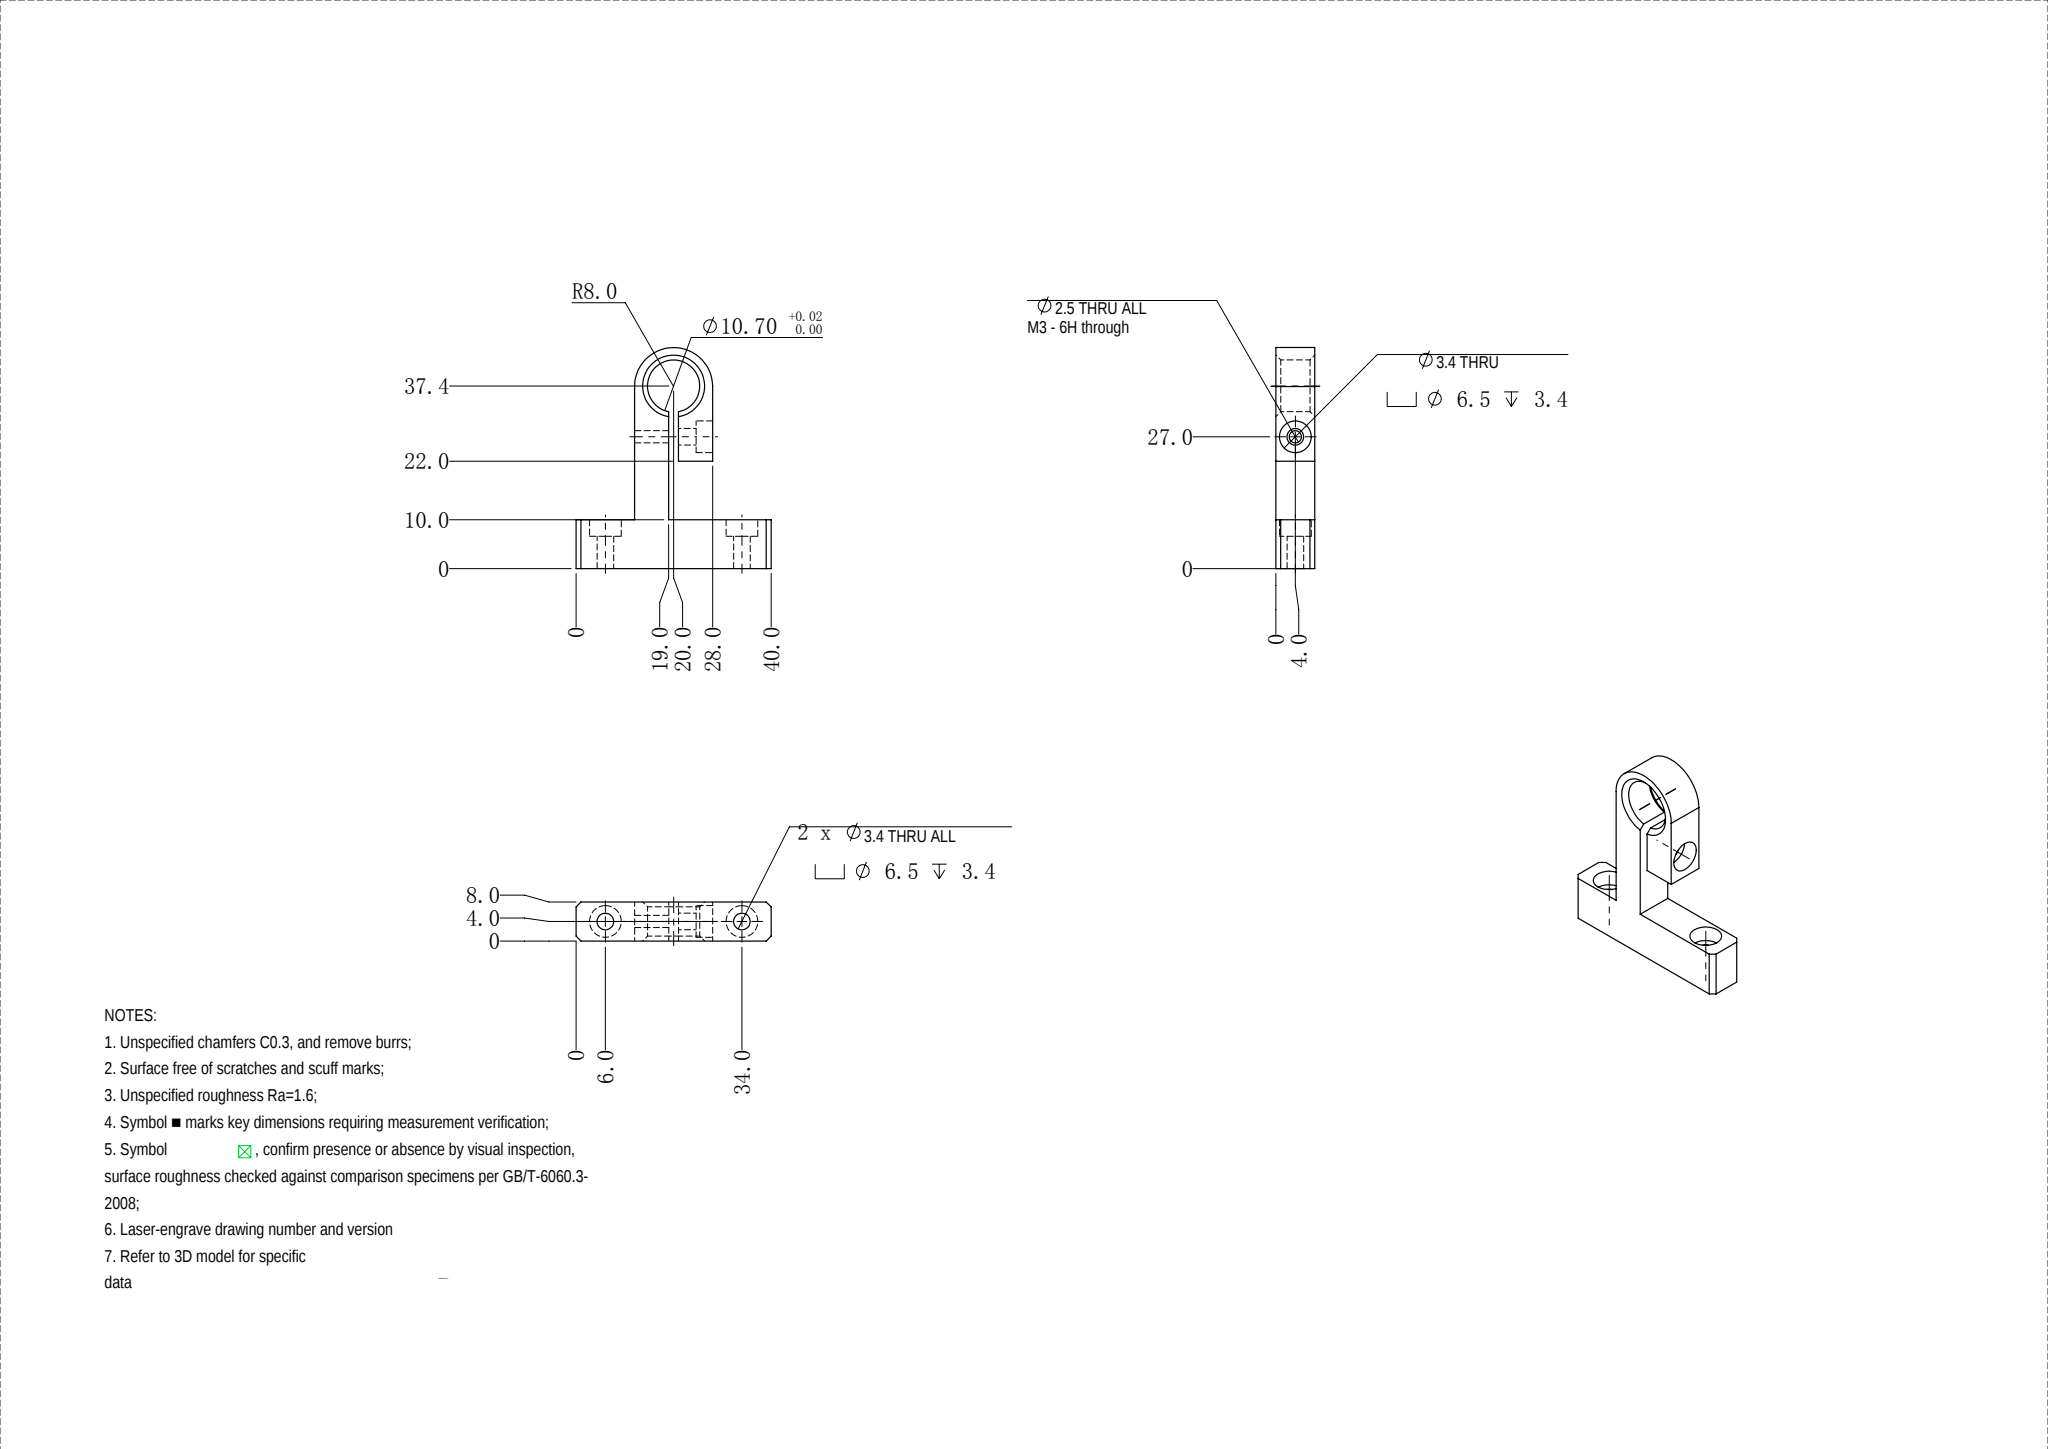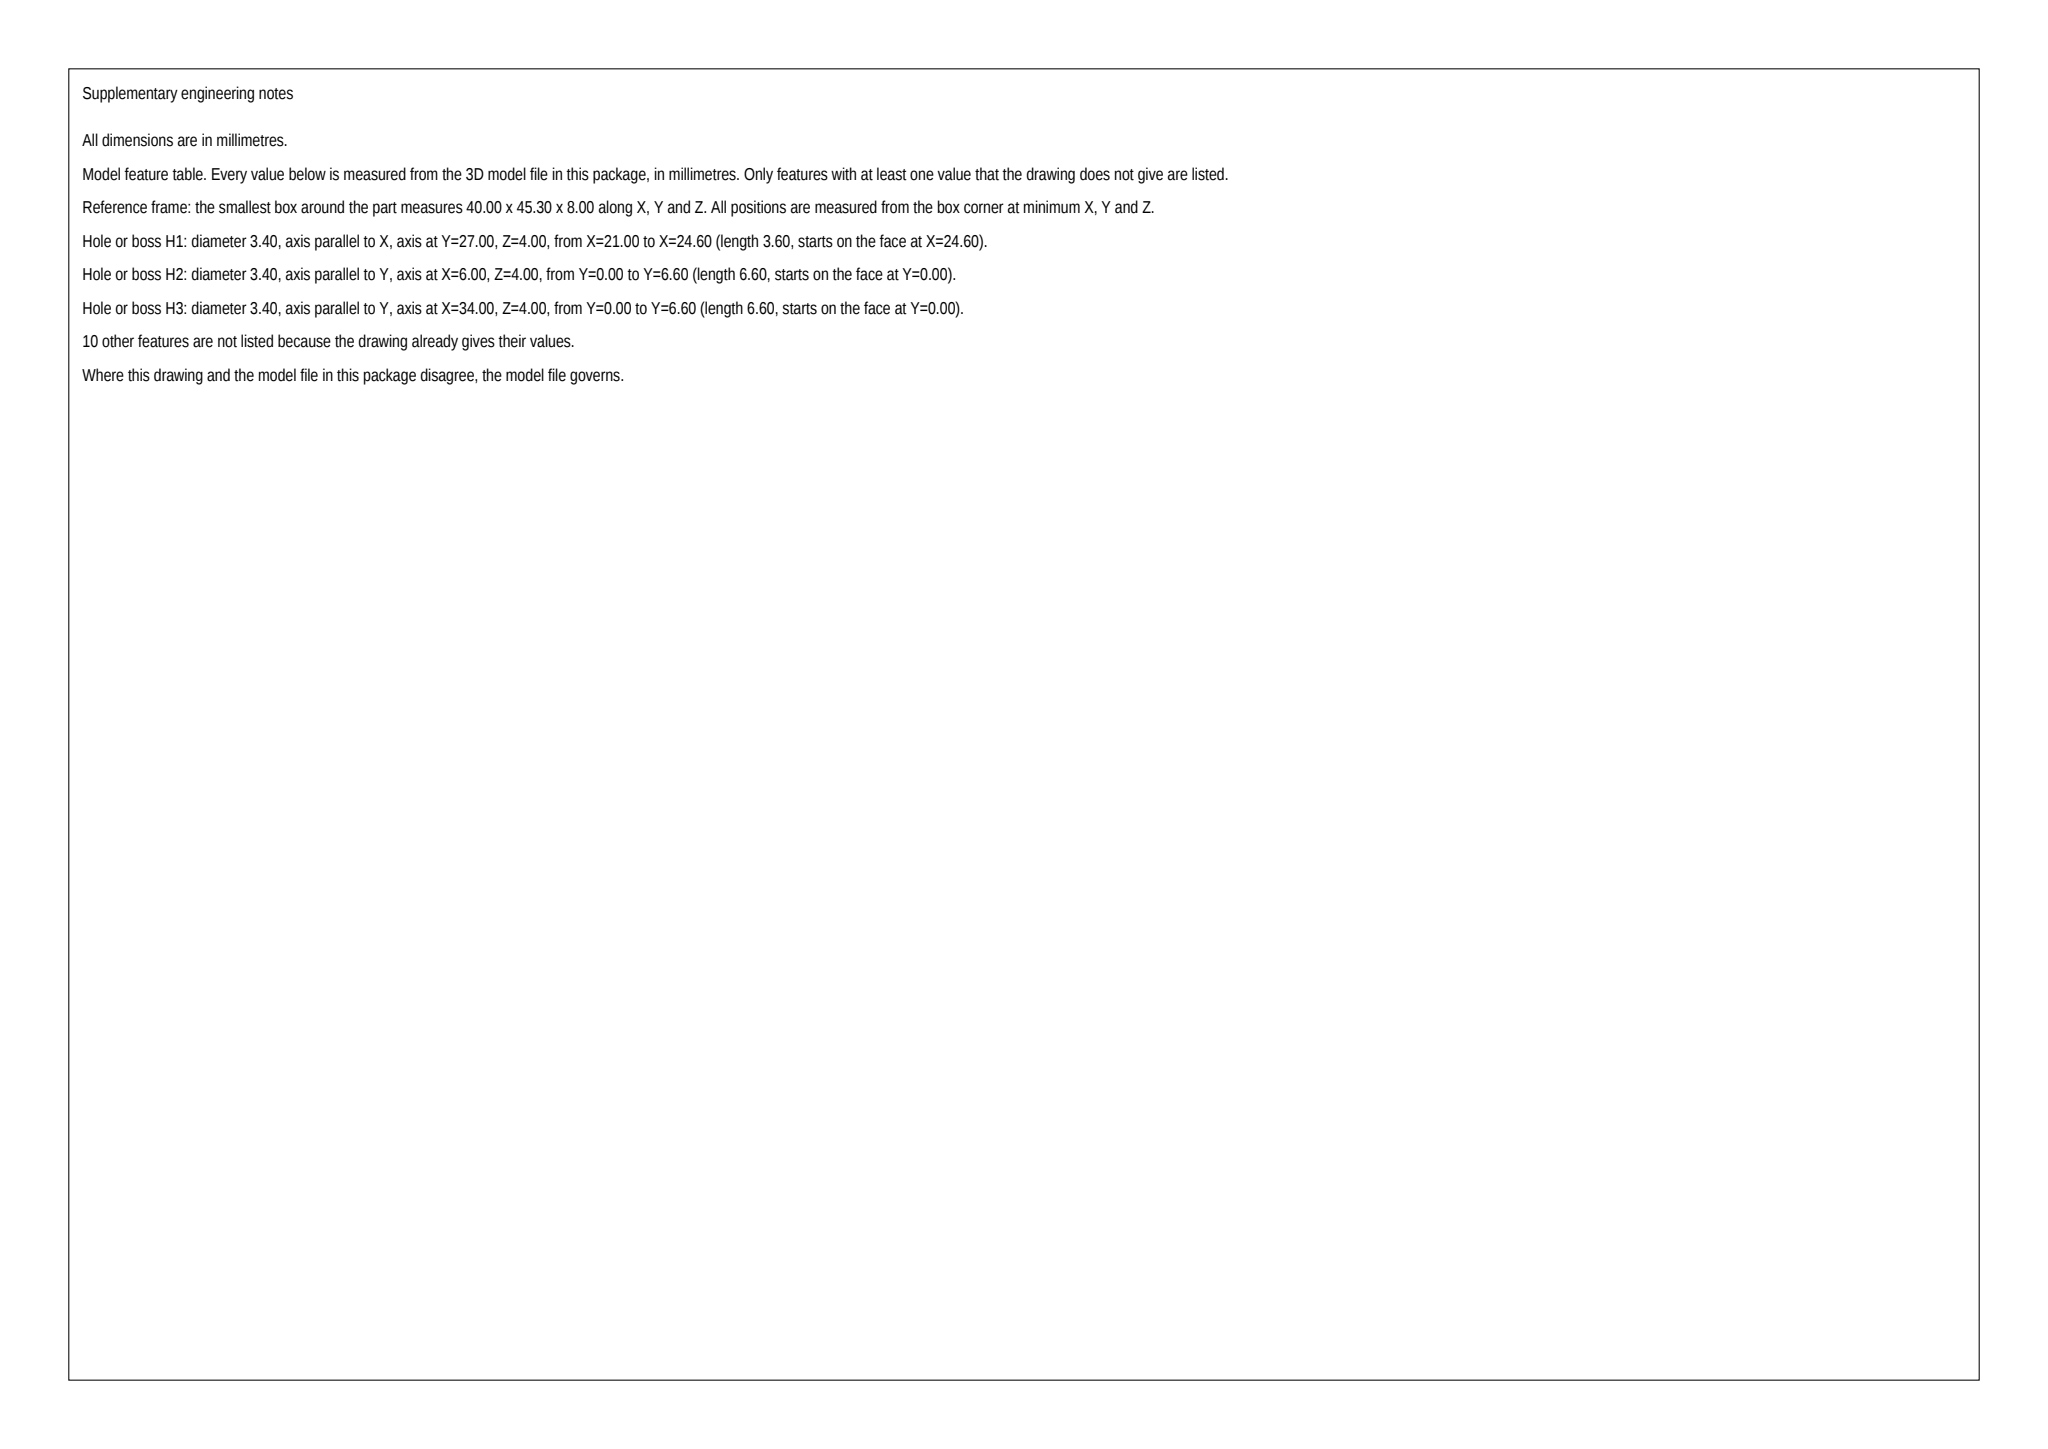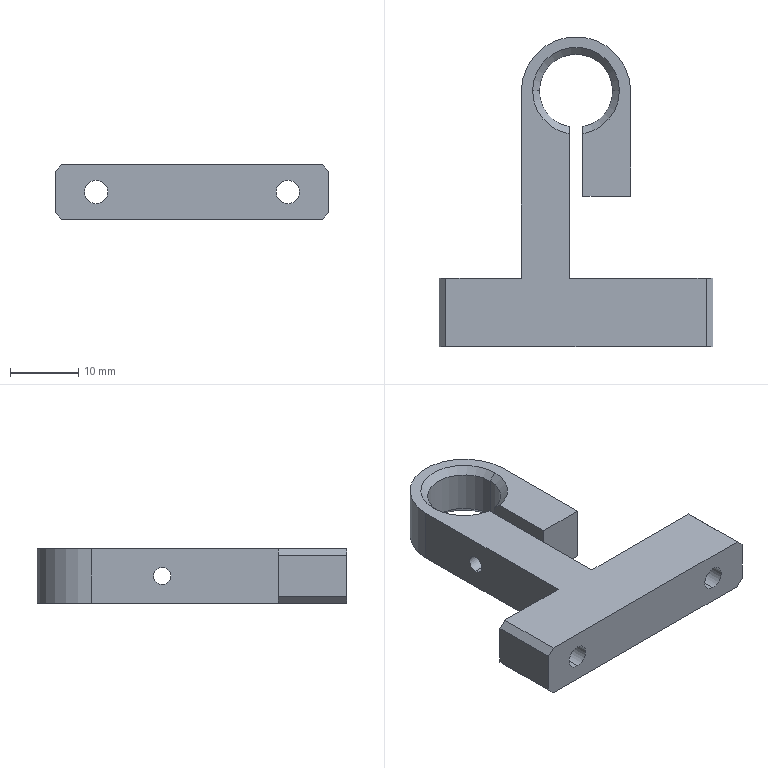Part | SolidWorks | mm | 1 solid | 43 faces | box 40 x 45.3 x 8 mm | volume 5175 mm3 | plane 19 | cylinder 18 | cone 6 | commonest cylinder face diameters 6.5 x6 3.4 x6 10.7 x3 2.5 x2 16 x1
Drawing notes:
OVERALL 40.0 X 45.3 X 8.0 | from the solid: bbox_xyz 40.0, 45.3, 8.0
2X Ø3.4 THRU / Ø6.5 CBORE DP 3.4 IN BASE: 6.0 & 34.0 FROM LH END, CL 4.0 FROM FRONT | from the solid: cyl dia 3.4 & 6.5 axis y at x=6.0 and x=34.0, z=4.0; x-planes 0.0/40.0